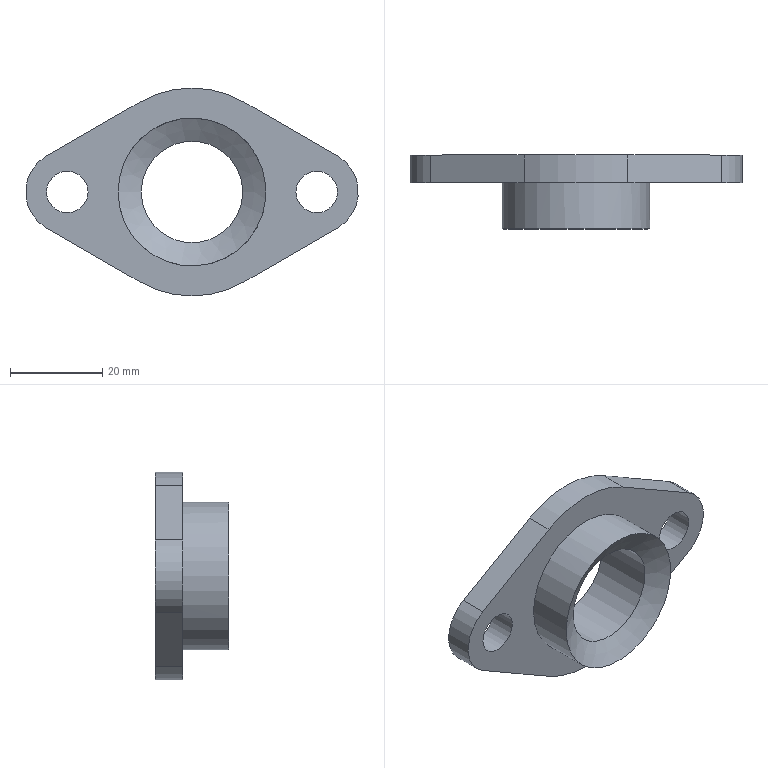Component | NX | PACKING_GLAND | 1 solid | 15 faces | volume 13660 mm3 | cylinder 8 | plane 6 | cone 1 | commonest cylinder face diameters 45 x2 18 x2 9 x2 32 x1 22 x1